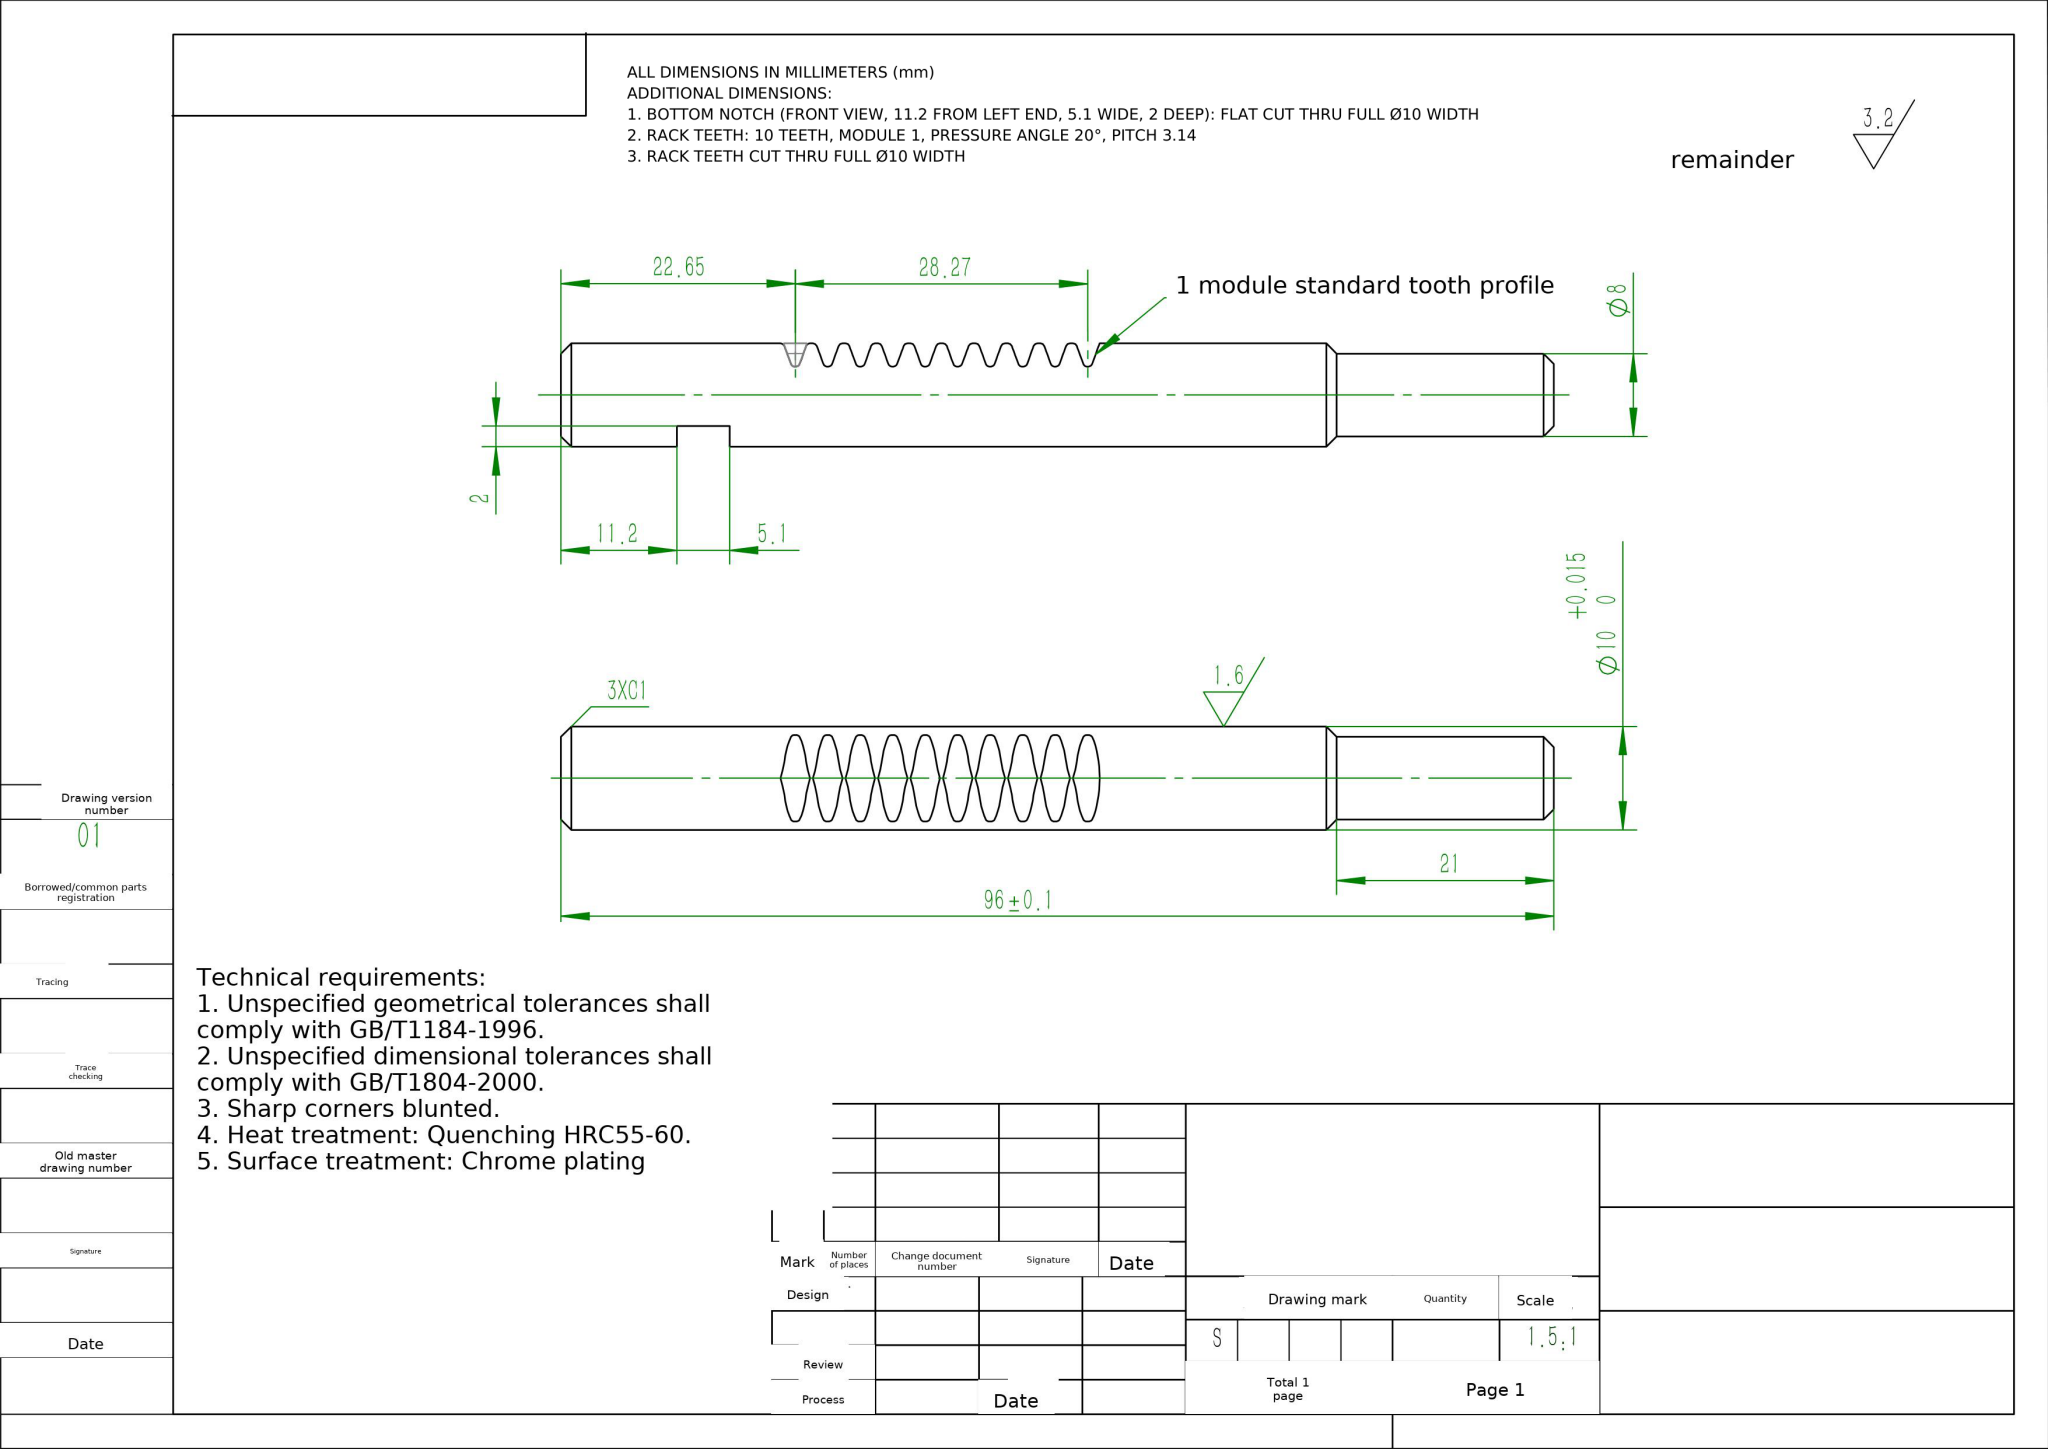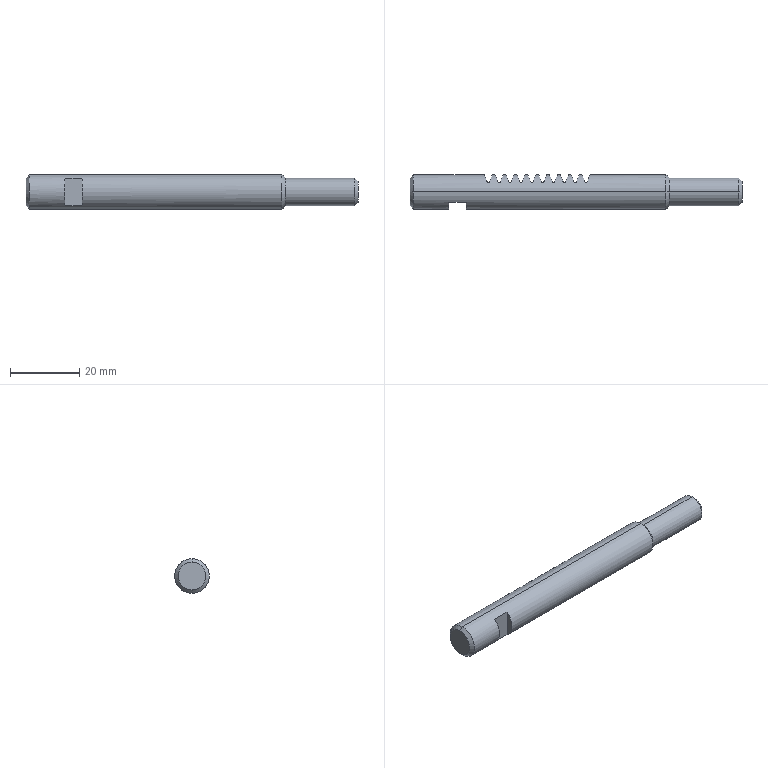Part | NX | mm | 1 solid | 84 faces | box 96 x 10 x 10 mm | volume 6674 mm3 | cylinder 43 | plane 35 | cone 6 | commonest cylinder face diameters 0.76 x20 0.8 x19 8 x2 10 x2